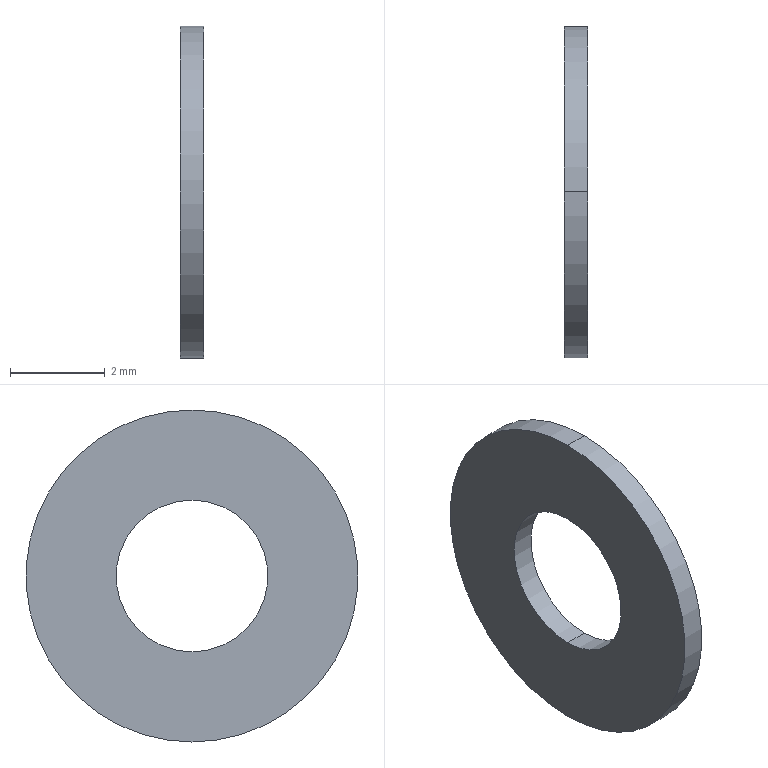Component | SolidWorks | plain washers--product grade c gb-3 | 1 solid | 6 faces | volume 15 mm3 | cylinder 4 | plane 2 | commonest cylinder face diameters 3.2 x2 7 x2